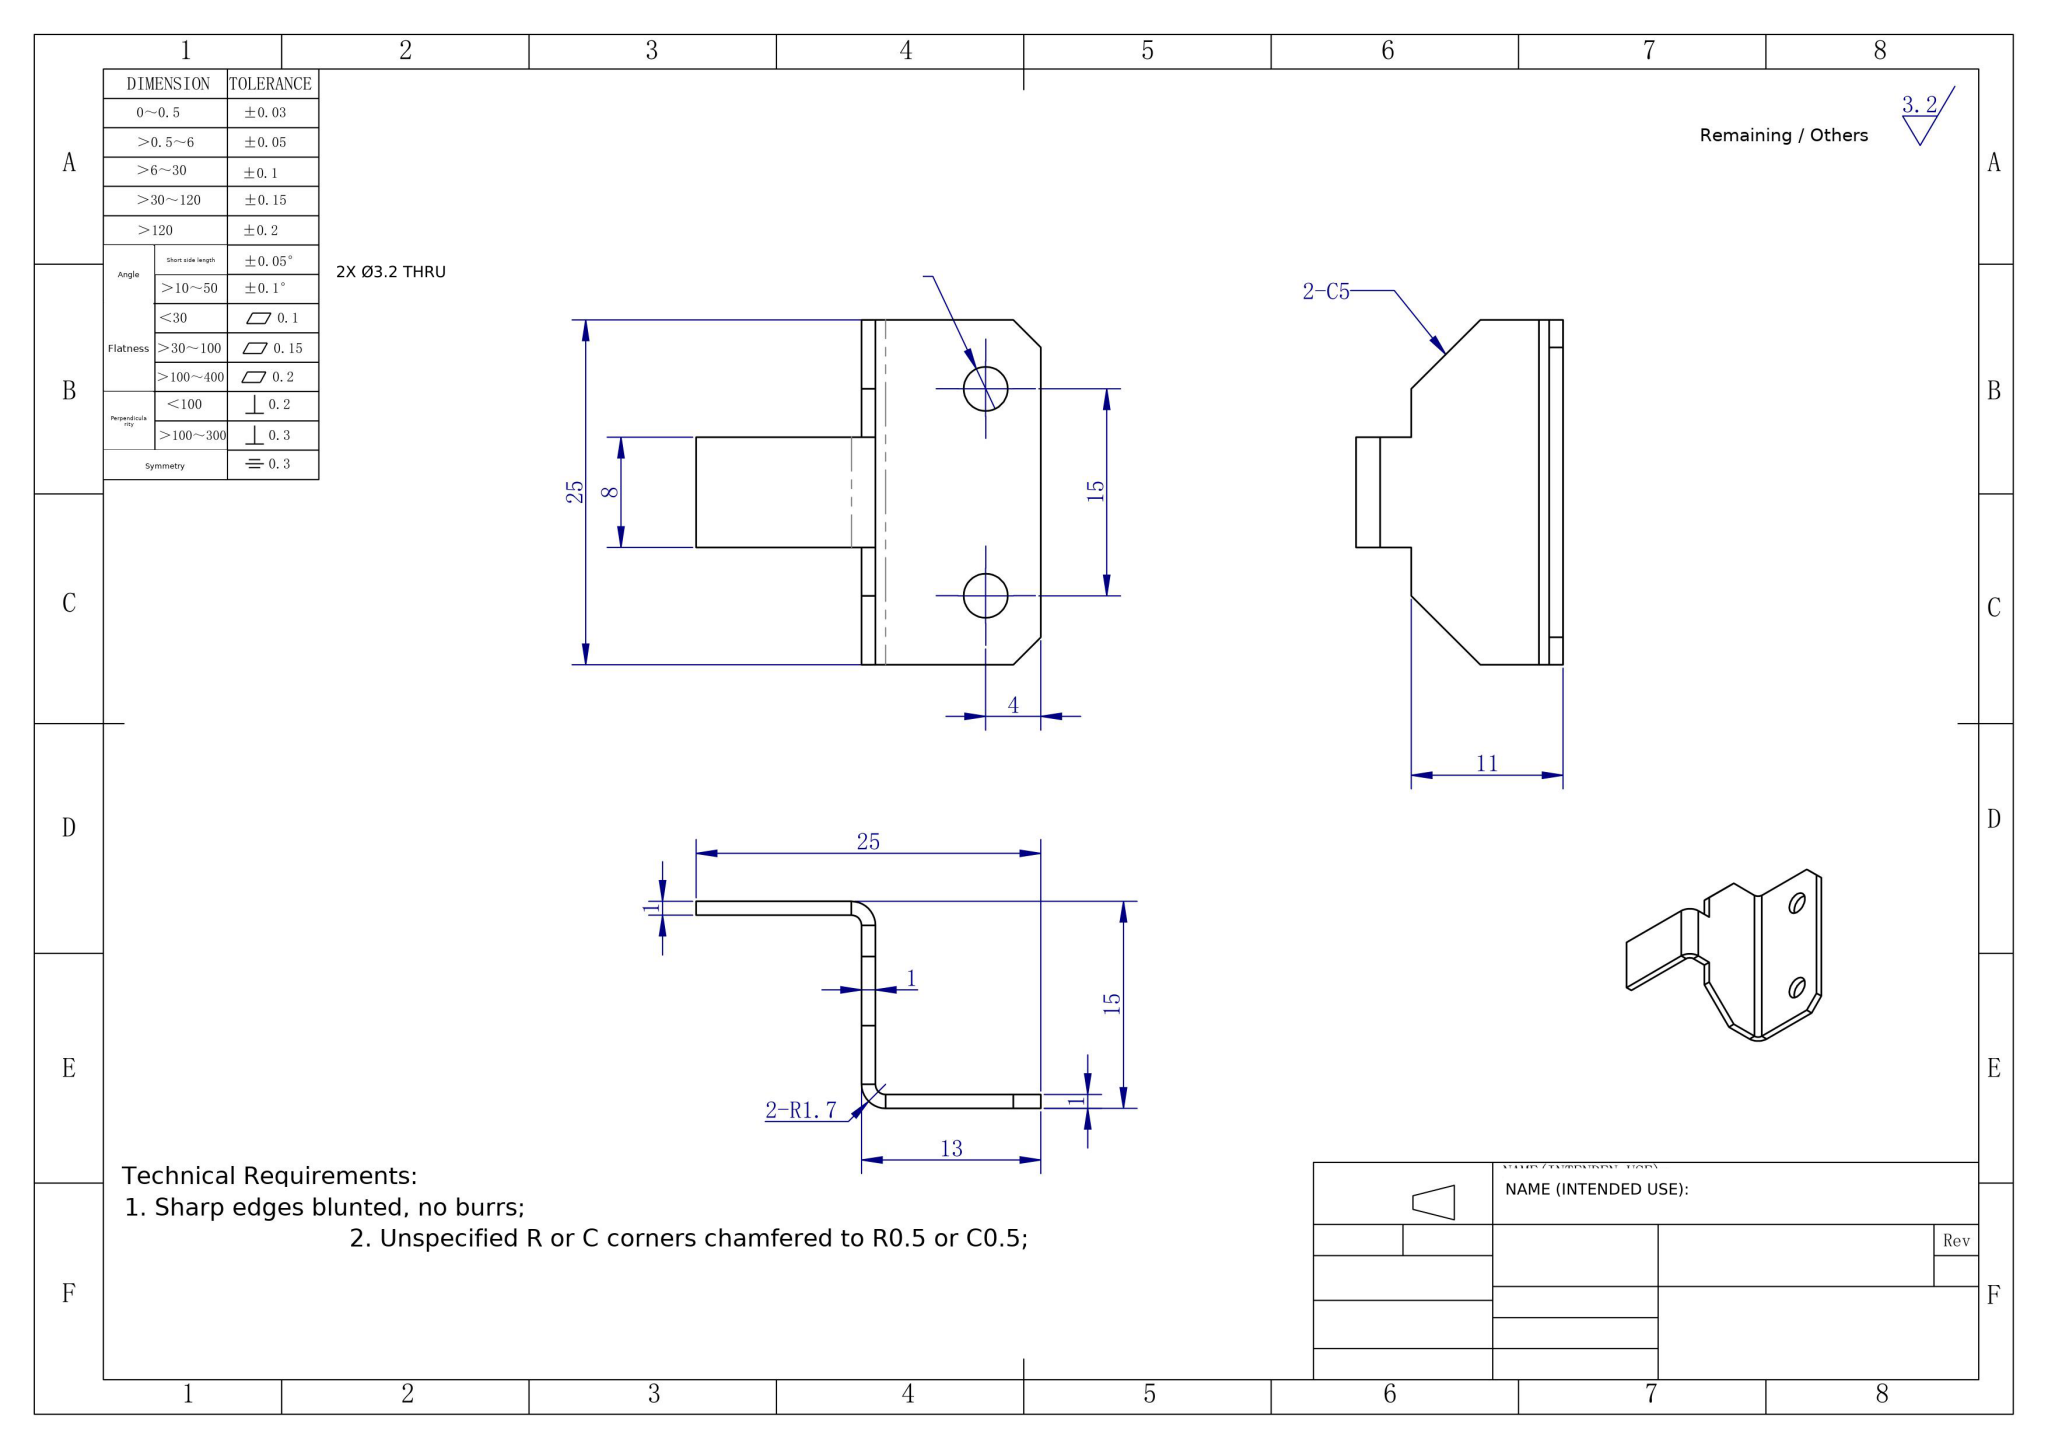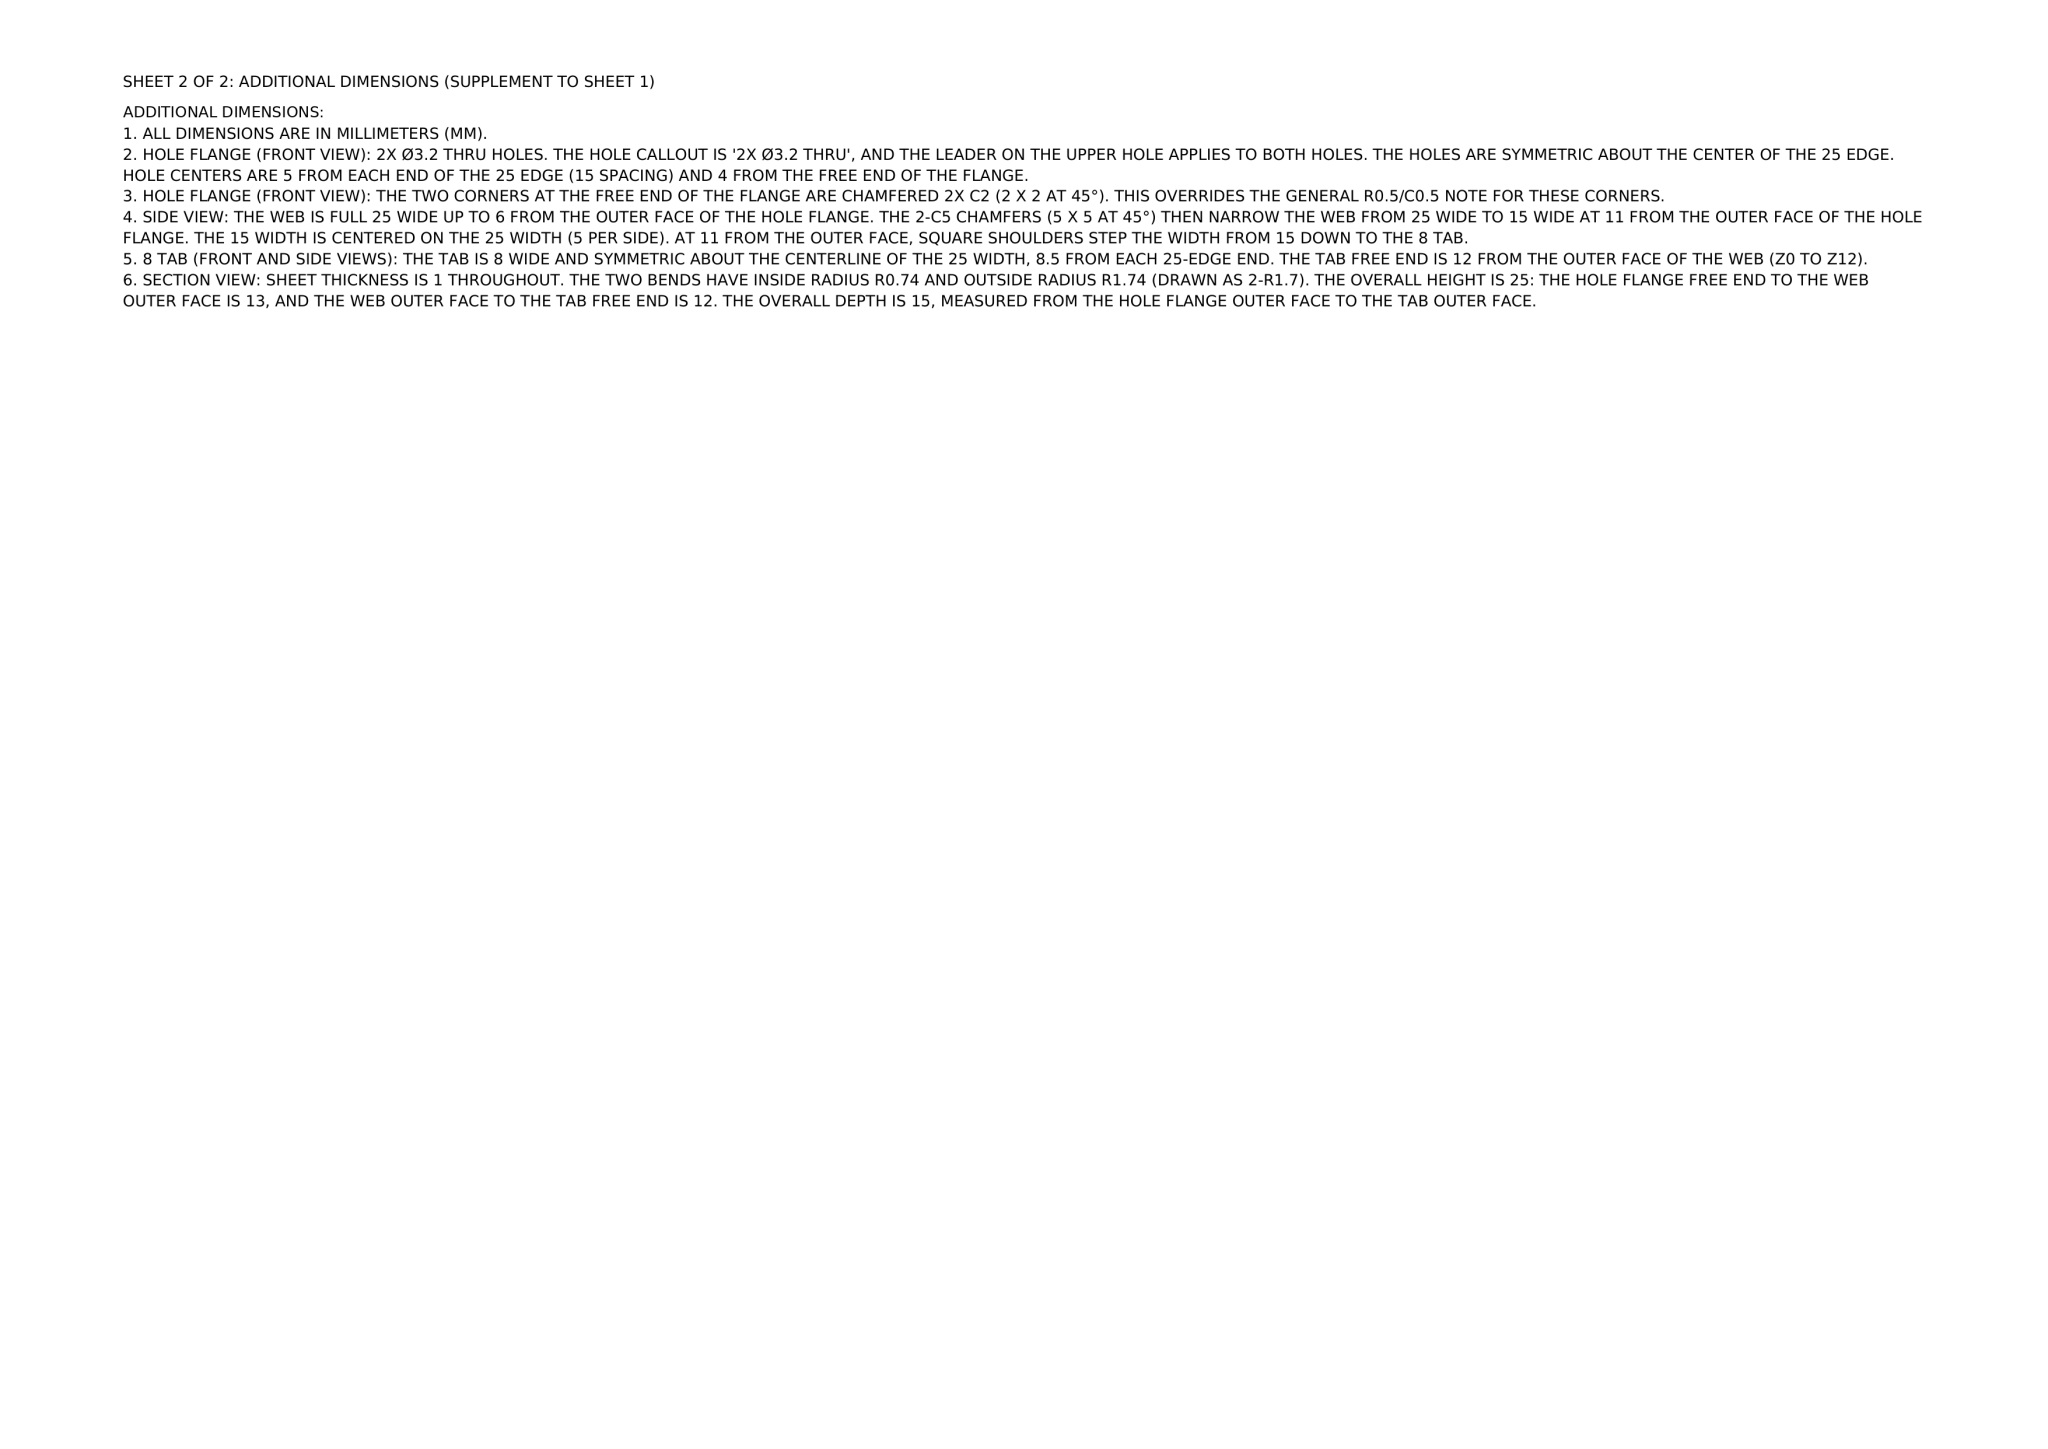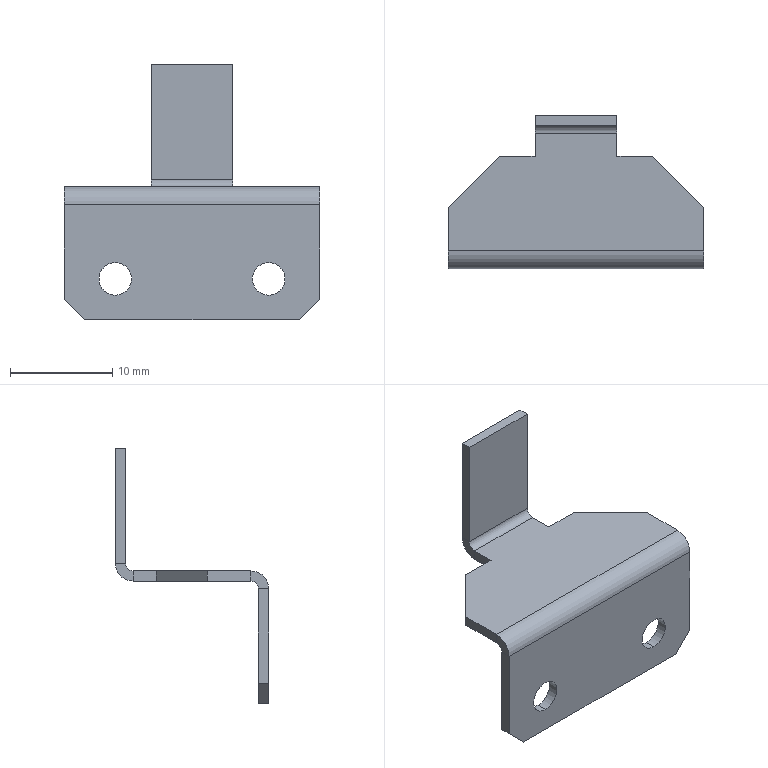Part | NX | mm | 1 solid | 34 faces | box 25 x 15 x 25 mm | volume 640 mm3 | plane 26 | cylinder 8 | commonest cylinder face diameters 3.2 x4 3.473 x2 1.473 x2